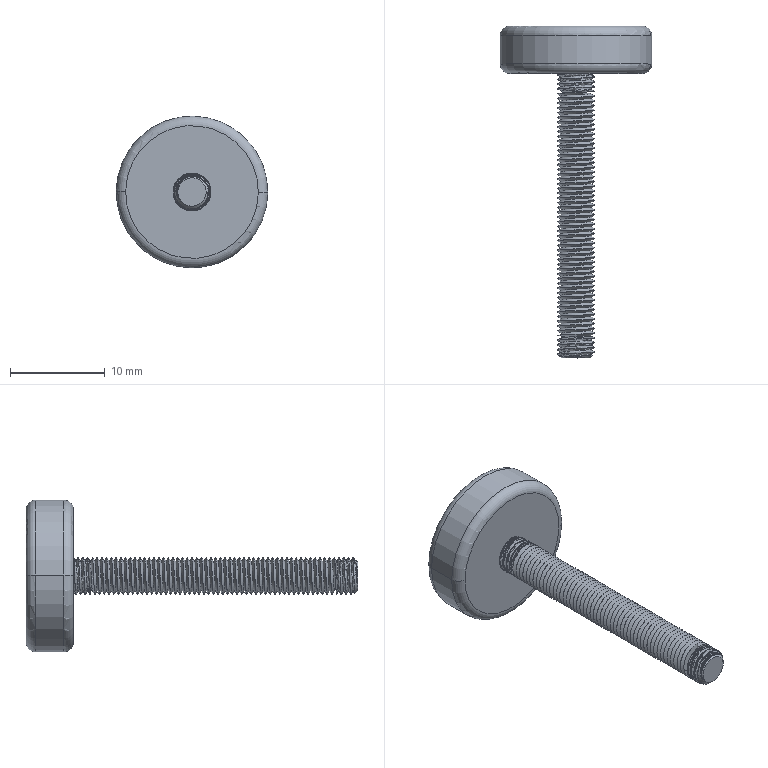Component | SolidWorks | Assembly5.1-1_ShortBoltM4.1-3 | 1 solid | 134 faces | volume 1286 mm3 | cylinder 122 | torus 4 | cone 3 | plane 3 | spline 2 | commonest cylinder face diameters 4 x120 16 x2